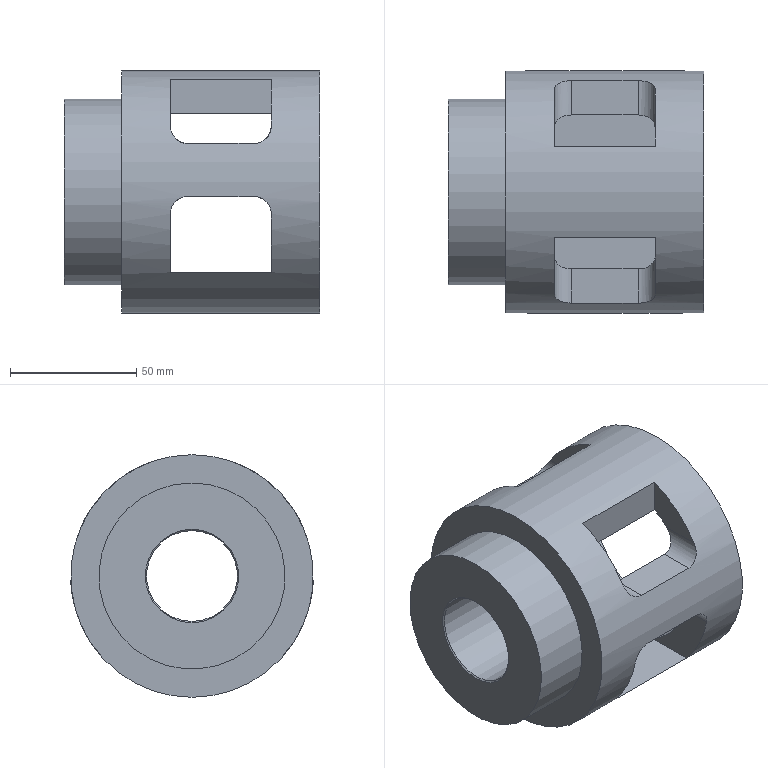Component | NX | BUSHING | 1 solid | 45 faces | volume 282225 mm3 | plane 26 | cylinder 18 | cone 1 | commonest cylinder face diameters 13.6 x8 8.5 x4 6 x2 96 x1 72 x1 73.6 x1 36 x1